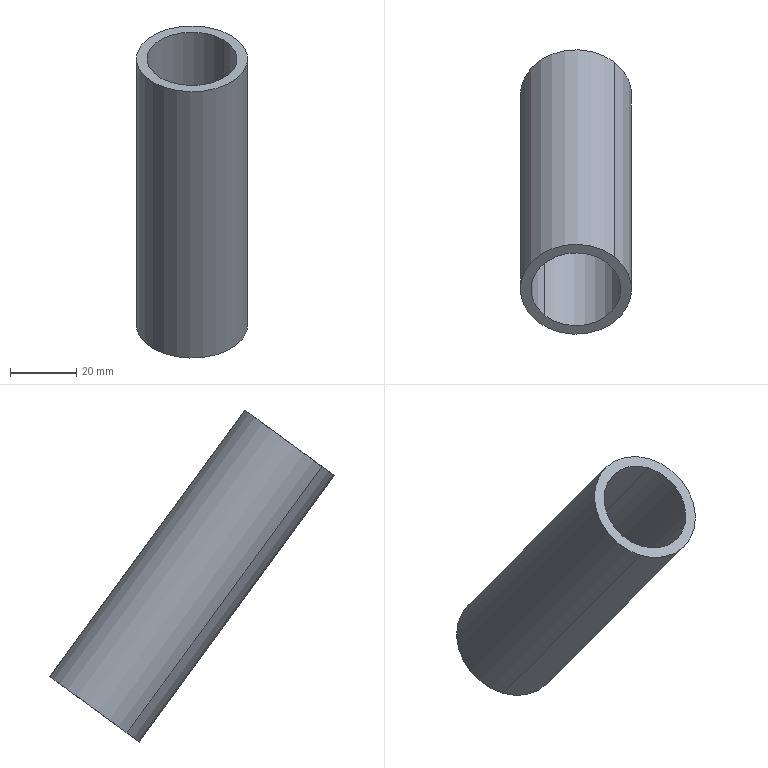Component | SolidWorks | circular tube_iso-10 | 1 solid | 6 faces | box 33.7 x 86.27 x 100.59 mm | volume 30662 mm3 | cylinder 4 | plane 2 | commonest cylinder face diameters 27.3 x2 33.7 x2
build123d program:
from build123d import *

# Parameters (mm, degrees)
SKETCH1_R      = 16.85
SKETCH1_R_2    = 13.65
BASEPIPE_DEPTH = 50


with BuildPart() as part:
    # Sketch1 → BasePipe (new, symmetric)
    with BuildSketch(Plane.XY):
        Circle(SKETCH1_R)
        Circle(SKETCH1_R_2, mode=Mode.SUBTRACT)
    extrude(amount=BASEPIPE_DEPTH, both=True)


solid = part.part

# Placed as in the assembly
solid = solid.moved(Location((-74, 669.859, 312.534), (36.21, 0, 6.454)))
STEP:
#1=COLOUR_RGB('',0.7922,0.8196,0.9333);
#2=FILL_AREA_STYLE_COLOUR('',#1);
#3=FILL_AREA_STYLE('',(#2));
#4=SURFACE_STYLE_FILL_AREA(#3);
#5=SURFACE_SIDE_STYLE('',(#4));
#6=SURFACE_STYLE_USAGE(.BOTH.,#5);
#7=PRESENTATION_STYLE_ASSIGNMENT((#6));
#8=CARTESIAN_POINT('',(-3.284,24.896,13.663));
#9=VERTEX_POINT('',#8);
#10=CARTESIAN_POINT('',(-2.542,25.523,14.122));
#11=VERTEX_POINT('',#10);
#12=CARTESIAN_POINT('',(-2.913,25.209,13.893));
#13=DIRECTION('',(0.,-0.5907,0.8069));
#14=DIRECTION('',(0.6902,0.5838,0.4275));
#15=AXIS2_PLACEMENT_3D('',#12,#13,#14);
#16=CIRCLE('',#15,0.5374);
#17=EDGE_CURVE('',#9,#11,#16,.T.);
#18=ORIENTED_EDGE('',*,*,#17,.T.);
#19=CARTESIAN_POINT('',(-2.542,27.849,10.946));
#20=VERTEX_POINT('',#19);
#21=CARTESIAN_POINT('',(-2.542,25.523,14.122));
#22=DIRECTION('',(-0.,0.5907,-0.8069));
#23=VECTOR('',#22,39.37);
#24=LINE('',#21,#23);
#25=EDGE_CURVE('',#11,#20,#24,.T.);
#26=ORIENTED_EDGE('',*,*,#25,.T.);
#27=CARTESIAN_POINT('',(-3.284,27.222,10.486));
#28=VERTEX_POINT('',#27);
#29=CARTESIAN_POINT('',(-2.913,27.535,10.716));
#30=DIRECTION('',(0.,-0.5907,0.8069));
#31=DIRECTION('',(0.6902,0.5838,0.4275));
#32=AXIS2_PLACEMENT_3D('',#29,#30,#31);
#33=CIRCLE('',#32,0.5374);
#34=EDGE_CURVE('',#28,#20,#33,.T.);
#35=ORIENTED_EDGE('',*,*,#34,.F.);
#36=CARTESIAN_POINT('',(-3.284,24.896,13.663));
#37=DIRECTION('',(-0.,0.5907,-0.8069));
#38=VECTOR('',#37,39.37);
#39=LINE('',#36,#38);
#40=EDGE_CURVE('',#9,#28,#39,.T.);
#41=ORIENTED_EDGE('',*,*,#40,.F.);
#42=EDGE_LOOP('',(#18,#26,#35,#41));
#43=FACE_OUTER_BOUND('',#42,.T.);
#44=CARTESIAN_POINT('',(-2.913,25.209,13.893));
#45=DIRECTION('',(-0.,0.5907,-0.8069));
#46=DIRECTION('',(-0.6902,-0.5838,-0.4275));
#47=AXIS2_PLACEMENT_3D('',#44,#45,#46);
#48=CYLINDRICAL_SURFACE('',#47,0.5374);
#49=ADVANCED_FACE('',(#43),#48,.F.);
#50=CARTESIAN_POINT('',(-2.456,25.597,14.176));
#51=VERTEX_POINT('',#50);
#52=CARTESIAN_POINT('',(-3.371,24.822,13.609));
#53=VERTEX_POINT('',#52);
#54=CARTESIAN_POINT('',(-2.913,25.209,13.893));
#55=DIRECTION('',(0.,-0.5907,0.8069));
#56=DIRECTION('',(0.6902,0.5838,0.4275));
#57=AXIS2_PLACEMENT_3D('',#54,#55,#56);
#58=CIRCLE('',#57,0.6634);
#59=EDGE_CURVE('',#51,#53,#58,.T.);
#60=ORIENTED_EDGE('',*,*,#59,.F.);
#61=CARTESIAN_POINT('',(-2.456,27.923,11.));
#62=VERTEX_POINT('',#61);
#63=CARTESIAN_POINT('',(-2.456,25.597,14.176));
#64=DIRECTION('',(-0.,0.5907,-0.8069));
#65=VECTOR('',#64,39.37);
#66=LINE('',#63,#65);
#67=EDGE_CURVE('',#51,#62,#66,.T.);
#68=ORIENTED_EDGE('',*,*,#67,.T.);
#69=CARTESIAN_POINT('',(-3.371,27.148,10.433));
#70=VERTEX_POINT('',#69);
#71=CARTESIAN_POINT('',(-2.913,27.535,10.716));
#72=DIRECTION('',(0.,-0.5907,0.8069));
#73=DIRECTION('',(0.6902,0.5838,0.4275));
#74=AXIS2_PLACEMENT_3D('',#71,#72,#73);
#75=CIRCLE('',#74,0.6634);
#76=EDGE_CURVE('',#62,#70,#75,.T.);
#77=ORIENTED_EDGE('',*,*,#76,.T.);
#78=CARTESIAN_POINT('',(-3.371,24.822,13.609));
#79=DIRECTION('',(-0.,0.5907,-0.8069));
#80=VECTOR('',#79,39.37);
#81=LINE('',#78,#80);
#82=EDGE_CURVE('',#53,#70,#81,.T.);
#83=ORIENTED_EDGE('',*,*,#82,.F.);
#84=EDGE_LOOP('',(#60,#68,#77,#83));
#85=FACE_OUTER_BOUND('',#84,.T.);
#86=CARTESIAN_POINT('',(-2.913,25.209,13.893));
#87=DIRECTION('',(-0.,0.5907,-0.8069));
#88=DIRECTION('',(-0.6902,-0.5838,-0.4275));
#89=AXIS2_PLACEMENT_3D('',#86,#87,#88);
#90=CYLINDRICAL_SURFACE('',#89,0.6634);
#91=ADVANCED_FACE('',(#85),#90,.T.);
#92=CARTESIAN_POINT('',(-2.913,25.209,13.893));
#93=DIRECTION('',(0.,-0.5907,0.8069));
#94=DIRECTION('',(0.6902,0.5838,0.4275));
#95=AXIS2_PLACEMENT_3D('',#92,#93,#94);
#96=CIRCLE('',#95,0.6634);
#97=EDGE_CURVE('',#53,#51,#96,.T.);
#98=ORIENTED_EDGE('',*,*,#97,.T.);
#99=ORIENTED_EDGE('',*,*,#59,.T.);
#100=EDGE_LOOP('',(#98,#99));
#101=FACE_OUTER_BOUND('',#100,.T.);
#102=ORIENTED_EDGE('',*,*,#17,.F.);
#103=CARTESIAN_POINT('',(-2.913,25.209,13.893));
#104=DIRECTION('',(0.,-0.5907,0.8069));
#105=DIRECTION('',(0.6902,0.5838,0.4275));
#106=AXIS2_PLACEMENT_3D('',#103,#104,#105);
#107=CIRCLE('',#106,0.5374);
#108=EDGE_CURVE('',#11,#9,#107,.T.);
#109=ORIENTED_EDGE('',*,*,#108,.F.);
#110=EDGE_LOOP('',(#102,#109));
#111=FACE_BOUND('',#110,.T.);
#112=CARTESIAN_POINT('',(-2.913,25.209,13.893));
#113=DIRECTION('',(0.,-0.5907,0.8069));
#114=DIRECTION('',(0.6902,0.5838,0.4275));
#115=AXIS2_PLACEMENT_3D('',#112,#113,#114);
#116=PLANE('',#115);
#117=ADVANCED_FACE('',(#101,#111),#116,.T.);
#118=CARTESIAN_POINT('',(-2.913,27.535,10.716));
#119=DIRECTION('',(0.,-0.5907,0.8069));
#120=DIRECTION('',(0.6902,0.5838,0.4275));
#121=AXIS2_PLACEMENT_3D('',#118,#119,#120);
#122=CIRCLE('',#121,0.6634);
#123=EDGE_CURVE('',#70,#62,#122,.T.);
#124=ORIENTED_EDGE('',*,*,#123,.F.);
#125=ORIENTED_EDGE('',*,*,#76,.F.);
#126=EDGE_LOOP('',(#124,#125));
#127=FACE_OUTER_BOUND('',#126,.T.);
#128=ORIENTED_EDGE('',*,*,#34,.T.);
#129=CARTESIAN_POINT('',(-2.913,27.535,10.716));
#130=DIRECTION('',(0.,-0.5907,0.8069));
#131=DIRECTION('',(0.6902,0.5838,0.4275));
#132=AXIS2_PLACEMENT_3D('',#129,#130,#131);
#133=CIRCLE('',#132,0.5374);
#134=EDGE_CURVE('',#20,#28,#133,.T.);
#135=ORIENTED_EDGE('',*,*,#134,.T.);
#136=EDGE_LOOP('',(#128,#135));
#137=FACE_BOUND('',#136,.T.);
#138=CARTESIAN_POINT('',(-2.913,27.535,10.716));
#139=DIRECTION('',(0.,-0.5907,0.8069));
#140=DIRECTION('',(0.6902,0.5838,0.4275));
#141=AXIS2_PLACEMENT_3D('',#138,#139,#140);
#142=PLANE('',#141);
#143=ADVANCED_FACE('',(#127,#137),#142,.F.);
#144=ORIENTED_EDGE('',*,*,#67,.F.);
#145=ORIENTED_EDGE('',*,*,#97,.F.);
#146=ORIENTED_EDGE('',*,*,#82,.T.);
#147=ORIENTED_EDGE('',*,*,#123,.T.);
#148=EDGE_LOOP('',(#144,#145,#146,#147));
#149=FACE_OUTER_BOUND('',#148,.T.);
#150=CARTESIAN_POINT('',(-2.913,25.209,13.893));
#151=DIRECTION('',(-0.,0.5907,-0.8069));
#152=DIRECTION('',(-0.6902,-0.5838,-0.4275));
#153=AXIS2_PLACEMENT_3D('',#150,#151,#152);
#154=CYLINDRICAL_SURFACE('',#153,0.6634);
#155=ADVANCED_FACE('',(#149),#154,.T.);
#156=ORIENTED_EDGE('',*,*,#25,.F.);
#157=ORIENTED_EDGE('',*,*,#108,.T.);
#158=ORIENTED_EDGE('',*,*,#40,.T.);
#159=ORIENTED_EDGE('',*,*,#134,.F.);
#160=EDGE_LOOP('',(#156,#157,#158,#159));
#161=FACE_OUTER_BOUND('',#160,.T.);
#162=CARTESIAN_POINT('',(-2.913,25.209,13.893));
#163=DIRECTION('',(-0.,0.5907,-0.8069));
#164=DIRECTION('',(-0.6902,-0.5838,-0.4275));
#165=AXIS2_PLACEMENT_3D('',#162,#163,#164);
#166=CYLINDRICAL_SURFACE('',#165,0.5374);
#167=ADVANCED_FACE('',(#161),#166,.F.);
#168=CLOSED_SHELL('',(#49,#91,#117,#143,#155,#167));
#169=MANIFOLD_SOLID_BREP('',#168);
#170=STYLED_ITEM('',(#7),#169);
#171=(LENGTH_UNIT()NAMED_UNIT(*)SI_UNIT($,.METRE.));
#172=LENGTH_MEASURE_WITH_UNIT(LENGTH_MEASURE(0.0254),#171);
#173=DIMENSIONAL_EXPONENTS(1.,0.,0.,0.,0.,0.,0.);
#174=(CONVERSION_BASED_UNIT('',#172)LENGTH_UNIT()NAMED_UNIT(#173));
#175=UNCERTAINTY_MEASURE_WITH_UNIT(LENGTH_MEASURE(0.00001),#174,'','');
#176=(NAMED_UNIT(*)PLANE_ANGLE_UNIT()SI_UNIT($,.RADIAN.));
#177=(NAMED_UNIT(*)SI_UNIT($,.STERADIAN.)SOLID_ANGLE_UNIT());
#178=(GEOMETRIC_REPRESENTATION_CONTEXT(3)GLOBAL_UNCERTAINTY_ASSIGNED_CONTEXT((#175))GLOBAL_UNIT_ASSIGNED_CONTEXT((#174,#176,#177))REPRESENTATION_CONTEXT('',''));
#179=MECHANICAL_DESIGN_GEOMETRIC_PRESENTATION_REPRESENTATION('',(#170),#178);
#180=CARTESIAN_POINT('',(0.,0.,0.));
#181=DIRECTION('',(0.,0.,1.));
#182=DIRECTION('',(1.,0.,0.));
#183=AXIS2_PLACEMENT_3D('',#180,#181,#182);
#184=(LENGTH_UNIT()NAMED_UNIT(*)SI_UNIT($,.METRE.));
#185=LENGTH_MEASURE_WITH_UNIT(LENGTH_MEASURE(0.0254),#184);
#186=DIMENSIONAL_EXPONENTS(1.,0.,0.,0.,0.,0.,0.);
#187=(CONVERSION_BASED_UNIT('',#185)LENGTH_UNIT()NAMED_UNIT(#186));
#188=UNCERTAINTY_MEASURE_WITH_UNIT(LENGTH_MEASURE(0.00001),#187,'','');
#189=(NAMED_UNIT(*)PLANE_ANGLE_UNIT()SI_UNIT($,.RADIAN.));
#190=(NAMED_UNIT(*)SI_UNIT($,.STERADIAN.)SOLID_ANGLE_UNIT());
#191=(GEOMETRIC_REPRESENTATION_CONTEXT(3)GLOBAL_UNCERTAINTY_ASSIGNED_CONTEXT((#188))GLOBAL_UNIT_ASSIGNED_CONTEXT((#187,#189,#190))REPRESENTATION_CONTEXT('',''));
#192=ADVANCED_BREP_SHAPE_REPRESENTATION('',(#169,#183),#191);
#193=PRESENTATION_LAYER_ASSIGNMENT('','',(#170));